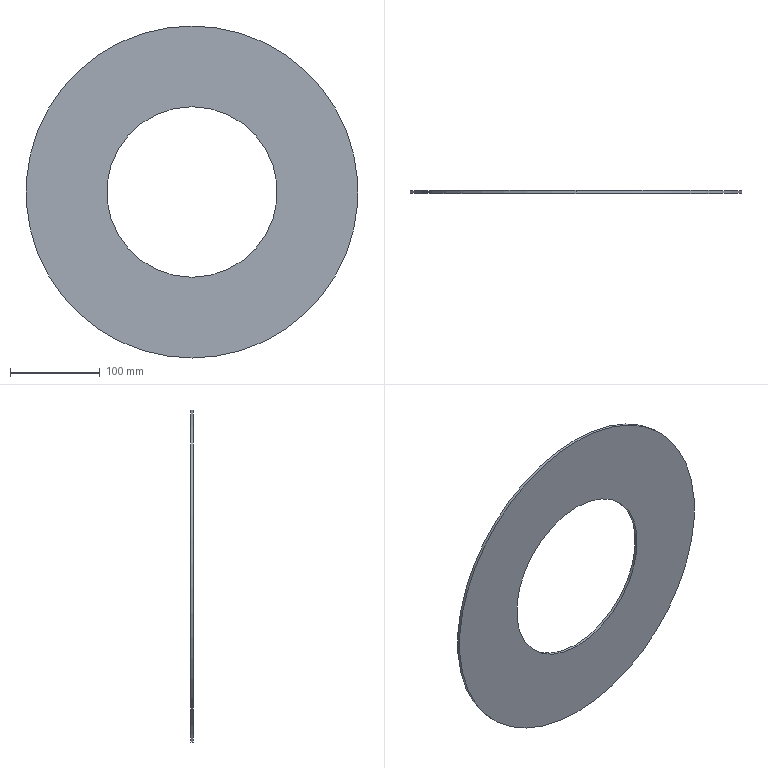Component | SolidWorks | YC1-250-03-01SliderAssembly-1_YC1-T-FCD-X8-1 | 1 solid | 6 faces | box 370 x 3 x 370 mm | volume 237504 mm3 | cylinder 4 | plane 2 | commonest cylinder face diameters 190 x2 370 x2 | material Plain Carbon Steel
STEP:
#1=COLOUR_RGB('',0.7922,0.8196,0.9333);
#2=FILL_AREA_STYLE_COLOUR('',#1);
#3=FILL_AREA_STYLE('',(#2));
#4=SURFACE_STYLE_FILL_AREA(#3);
#5=SURFACE_SIDE_STYLE('',(#4));
#6=SURFACE_STYLE_USAGE(.BOTH.,#5);
#7=PRESENTATION_STYLE_ASSIGNMENT((#6));
#8=CARTESIAN_POINT('',(0.1124,94.419,3.827));
#9=VERTEX_POINT('',#8);
#10=CARTESIAN_POINT('',(0.1124,94.419,-3.653));
#11=VERTEX_POINT('',#10);
#12=CARTESIAN_POINT('',(0.1124,94.419,0.08684));
#13=DIRECTION('',(0.,-1.,0.));
#14=DIRECTION('',(0.,0.,-1.));
#15=AXIS2_PLACEMENT_3D('',#12,#13,#14);
#16=CIRCLE('',#15,3.74);
#17=EDGE_CURVE('',#9,#11,#16,.T.);
#18=ORIENTED_EDGE('',*,*,#17,.F.);
#19=CARTESIAN_POINT('',(0.1124,94.301,3.827));
#20=VERTEX_POINT('',#19);
#21=CARTESIAN_POINT('',(0.1124,94.419,3.827));
#22=DIRECTION('',(0.,-1.,0.));
#23=VECTOR('',#22,39.37);
#24=LINE('',#21,#23);
#25=EDGE_CURVE('',#9,#20,#24,.T.);
#26=ORIENTED_EDGE('',*,*,#25,.T.);
#27=CARTESIAN_POINT('',(0.1124,94.301,-3.653));
#28=VERTEX_POINT('',#27);
#29=CARTESIAN_POINT('',(0.1124,94.301,0.08684));
#30=DIRECTION('',(0.,1.,0.));
#31=DIRECTION('',(0.,0.,-1.));
#32=AXIS2_PLACEMENT_3D('',#29,#30,#31);
#33=CIRCLE('',#32,3.74);
#34=EDGE_CURVE('',#28,#20,#33,.T.);
#35=ORIENTED_EDGE('',*,*,#34,.F.);
#36=CARTESIAN_POINT('',(0.1124,94.419,-3.653));
#37=DIRECTION('',(0.,-1.,0.));
#38=VECTOR('',#37,39.37);
#39=LINE('',#36,#38);
#40=EDGE_CURVE('',#11,#28,#39,.T.);
#41=ORIENTED_EDGE('',*,*,#40,.F.);
#42=EDGE_LOOP('',(#18,#26,#35,#41));
#43=FACE_OUTER_BOUND('',#42,.T.);
#44=CARTESIAN_POINT('',(0.1124,94.419,0.08684));
#45=DIRECTION('',(0.,-1.,0.));
#46=DIRECTION('',(0.,0.,-1.));
#47=AXIS2_PLACEMENT_3D('',#44,#45,#46);
#48=CYLINDRICAL_SURFACE('',#47,3.74);
#49=ADVANCED_FACE('',(#43),#48,.F.);
#50=CARTESIAN_POINT('',(0.1124,94.419,7.37));
#51=VERTEX_POINT('',#50);
#52=CARTESIAN_POINT('',(0.1124,94.419,-7.197));
#53=VERTEX_POINT('',#52);
#54=CARTESIAN_POINT('',(0.1124,94.419,0.08684));
#55=DIRECTION('',(0.,1.,0.));
#56=DIRECTION('',(0.,0.,-1.));
#57=AXIS2_PLACEMENT_3D('',#54,#55,#56);
#58=CIRCLE('',#57,7.283);
#59=EDGE_CURVE('',#51,#53,#58,.T.);
#60=ORIENTED_EDGE('',*,*,#59,.F.);
#61=CARTESIAN_POINT('',(0.1124,94.301,7.37));
#62=VERTEX_POINT('',#61);
#63=CARTESIAN_POINT('',(0.1124,94.419,7.37));
#64=DIRECTION('',(0.,-1.,0.));
#65=VECTOR('',#64,39.37);
#66=LINE('',#63,#65);
#67=EDGE_CURVE('',#51,#62,#66,.T.);
#68=ORIENTED_EDGE('',*,*,#67,.T.);
#69=CARTESIAN_POINT('',(0.1124,94.301,-7.197));
#70=VERTEX_POINT('',#69);
#71=CARTESIAN_POINT('',(0.1124,94.301,0.08684));
#72=DIRECTION('',(0.,1.,0.));
#73=DIRECTION('',(0.,0.,-1.));
#74=AXIS2_PLACEMENT_3D('',#71,#72,#73);
#75=CIRCLE('',#74,7.283);
#76=EDGE_CURVE('',#62,#70,#75,.T.);
#77=ORIENTED_EDGE('',*,*,#76,.T.);
#78=CARTESIAN_POINT('',(0.1124,94.419,-7.197));
#79=DIRECTION('',(0.,-1.,0.));
#80=VECTOR('',#79,39.37);
#81=LINE('',#78,#80);
#82=EDGE_CURVE('',#53,#70,#81,.T.);
#83=ORIENTED_EDGE('',*,*,#82,.F.);
#84=EDGE_LOOP('',(#60,#68,#77,#83));
#85=FACE_OUTER_BOUND('',#84,.T.);
#86=CARTESIAN_POINT('',(0.1124,94.419,0.08684));
#87=DIRECTION('',(0.,-1.,0.));
#88=DIRECTION('',(0.,0.,-1.));
#89=AXIS2_PLACEMENT_3D('',#86,#87,#88);
#90=CYLINDRICAL_SURFACE('',#89,7.283);
#91=ADVANCED_FACE('',(#85),#90,.T.);
#92=CARTESIAN_POINT('',(0.1124,94.419,0.08684));
#93=DIRECTION('',(0.,-1.,0.));
#94=DIRECTION('',(0.,0.,-1.));
#95=AXIS2_PLACEMENT_3D('',#92,#93,#94);
#96=CIRCLE('',#95,3.74);
#97=EDGE_CURVE('',#11,#9,#96,.T.);
#98=ORIENTED_EDGE('',*,*,#97,.T.);
#99=ORIENTED_EDGE('',*,*,#17,.T.);
#100=EDGE_LOOP('',(#98,#99));
#101=FACE_BOUND('',#100,.T.);
#102=CARTESIAN_POINT('',(0.1124,94.419,0.08684));
#103=DIRECTION('',(0.,1.,0.));
#104=DIRECTION('',(0.,0.,-1.));
#105=AXIS2_PLACEMENT_3D('',#102,#103,#104);
#106=CIRCLE('',#105,7.283);
#107=EDGE_CURVE('',#53,#51,#106,.T.);
#108=ORIENTED_EDGE('',*,*,#107,.T.);
#109=ORIENTED_EDGE('',*,*,#59,.T.);
#110=EDGE_LOOP('',(#108,#109));
#111=FACE_OUTER_BOUND('',#110,.T.);
#112=CARTESIAN_POINT('',(0.1124,94.419,0.08684));
#113=DIRECTION('',(0.,1.,0.));
#114=DIRECTION('',(0.,0.,1.));
#115=AXIS2_PLACEMENT_3D('',#112,#113,#114);
#116=PLANE('',#115);
#117=ADVANCED_FACE('',(#101,#111),#116,.T.);
#118=ORIENTED_EDGE('',*,*,#25,.F.);
#119=ORIENTED_EDGE('',*,*,#97,.F.);
#120=ORIENTED_EDGE('',*,*,#40,.T.);
#121=CARTESIAN_POINT('',(0.1124,94.301,0.08684));
#122=DIRECTION('',(0.,1.,0.));
#123=DIRECTION('',(0.,0.,-1.));
#124=AXIS2_PLACEMENT_3D('',#121,#122,#123);
#125=CIRCLE('',#124,3.74);
#126=EDGE_CURVE('',#20,#28,#125,.T.);
#127=ORIENTED_EDGE('',*,*,#126,.F.);
#128=EDGE_LOOP('',(#118,#119,#120,#127));
#129=FACE_OUTER_BOUND('',#128,.T.);
#130=CARTESIAN_POINT('',(0.1124,94.419,0.08684));
#131=DIRECTION('',(0.,-1.,0.));
#132=DIRECTION('',(0.,0.,-1.));
#133=AXIS2_PLACEMENT_3D('',#130,#131,#132);
#134=CYLINDRICAL_SURFACE('',#133,3.74);
#135=ADVANCED_FACE('',(#129),#134,.F.);
#136=ORIENTED_EDGE('',*,*,#67,.F.);
#137=ORIENTED_EDGE('',*,*,#107,.F.);
#138=ORIENTED_EDGE('',*,*,#82,.T.);
#139=CARTESIAN_POINT('',(0.1124,94.301,0.08684));
#140=DIRECTION('',(0.,1.,0.));
#141=DIRECTION('',(0.,0.,-1.));
#142=AXIS2_PLACEMENT_3D('',#139,#140,#141);
#143=CIRCLE('',#142,7.283);
#144=EDGE_CURVE('',#70,#62,#143,.T.);
#145=ORIENTED_EDGE('',*,*,#144,.T.);
#146=EDGE_LOOP('',(#136,#137,#138,#145));
#147=FACE_OUTER_BOUND('',#146,.T.);
#148=CARTESIAN_POINT('',(0.1124,94.419,0.08684));
#149=DIRECTION('',(0.,-1.,0.));
#150=DIRECTION('',(0.,0.,-1.));
#151=AXIS2_PLACEMENT_3D('',#148,#149,#150);
#152=CYLINDRICAL_SURFACE('',#151,7.283);
#153=ADVANCED_FACE('',(#147),#152,.T.);
#154=ORIENTED_EDGE('',*,*,#34,.T.);
#155=ORIENTED_EDGE('',*,*,#126,.T.);
#156=EDGE_LOOP('',(#154,#155));
#157=FACE_BOUND('',#156,.T.);
#158=ORIENTED_EDGE('',*,*,#144,.F.);
#159=ORIENTED_EDGE('',*,*,#76,.F.);
#160=EDGE_LOOP('',(#158,#159));
#161=FACE_OUTER_BOUND('',#160,.T.);
#162=CARTESIAN_POINT('',(0.1124,94.301,0.08684));
#163=DIRECTION('',(0.,1.,0.));
#164=DIRECTION('',(0.,0.,1.));
#165=AXIS2_PLACEMENT_3D('',#162,#163,#164);
#166=PLANE('',#165);
#167=ADVANCED_FACE('',(#157,#161),#166,.F.);
#168=CLOSED_SHELL('',(#49,#91,#117,#135,#153,#167));
#169=MANIFOLD_SOLID_BREP('',#168);
#170=STYLED_ITEM('',(#7),#169);
#171=(LENGTH_UNIT()NAMED_UNIT(*)SI_UNIT($,.METRE.));
#172=LENGTH_MEASURE_WITH_UNIT(LENGTH_MEASURE(0.0254),#171);
#173=DIMENSIONAL_EXPONENTS(1.,0.,0.,0.,0.,0.,0.);
#174=(CONVERSION_BASED_UNIT('',#172)LENGTH_UNIT()NAMED_UNIT(#173));
#175=UNCERTAINTY_MEASURE_WITH_UNIT(LENGTH_MEASURE(0.00001),#174,'','');
#176=(NAMED_UNIT(*)PLANE_ANGLE_UNIT()SI_UNIT($,.RADIAN.));
#177=(NAMED_UNIT(*)SI_UNIT($,.STERADIAN.)SOLID_ANGLE_UNIT());
#178=(GEOMETRIC_REPRESENTATION_CONTEXT(3)GLOBAL_UNCERTAINTY_ASSIGNED_CONTEXT((#175))GLOBAL_UNIT_ASSIGNED_CONTEXT((#174,#176,#177))REPRESENTATION_CONTEXT('',''));
#179=MECHANICAL_DESIGN_GEOMETRIC_PRESENTATION_REPRESENTATION('',(#170),#178);
#180=CARTESIAN_POINT('',(0.,0.,0.));
#181=DIRECTION('',(0.,0.,1.));
#182=DIRECTION('',(1.,0.,0.));
#183=AXIS2_PLACEMENT_3D('',#180,#181,#182);
#184=(LENGTH_UNIT()NAMED_UNIT(*)SI_UNIT($,.METRE.));
#185=LENGTH_MEASURE_WITH_UNIT(LENGTH_MEASURE(0.0254),#184);
#186=DIMENSIONAL_EXPONENTS(1.,0.,0.,0.,0.,0.,0.);
#187=(CONVERSION_BASED_UNIT('',#185)LENGTH_UNIT()NAMED_UNIT(#186));
#188=UNCERTAINTY_MEASURE_WITH_UNIT(LENGTH_MEASURE(0.00001),#187,'','');
#189=(NAMED_UNIT(*)PLANE_ANGLE_UNIT()SI_UNIT($,.RADIAN.));
#190=(NAMED_UNIT(*)SI_UNIT($,.STERADIAN.)SOLID_ANGLE_UNIT());
#191=(GEOMETRIC_REPRESENTATION_CONTEXT(3)GLOBAL_UNCERTAINTY_ASSIGNED_CONTEXT((#188))GLOBAL_UNIT_ASSIGNED_CONTEXT((#187,#189,#190))REPRESENTATION_CONTEXT('',''));
#192=ADVANCED_BREP_SHAPE_REPRESENTATION('',(#169,#183),#191);
#193=PRESENTATION_LAYER_ASSIGNMENT('','',(#170));